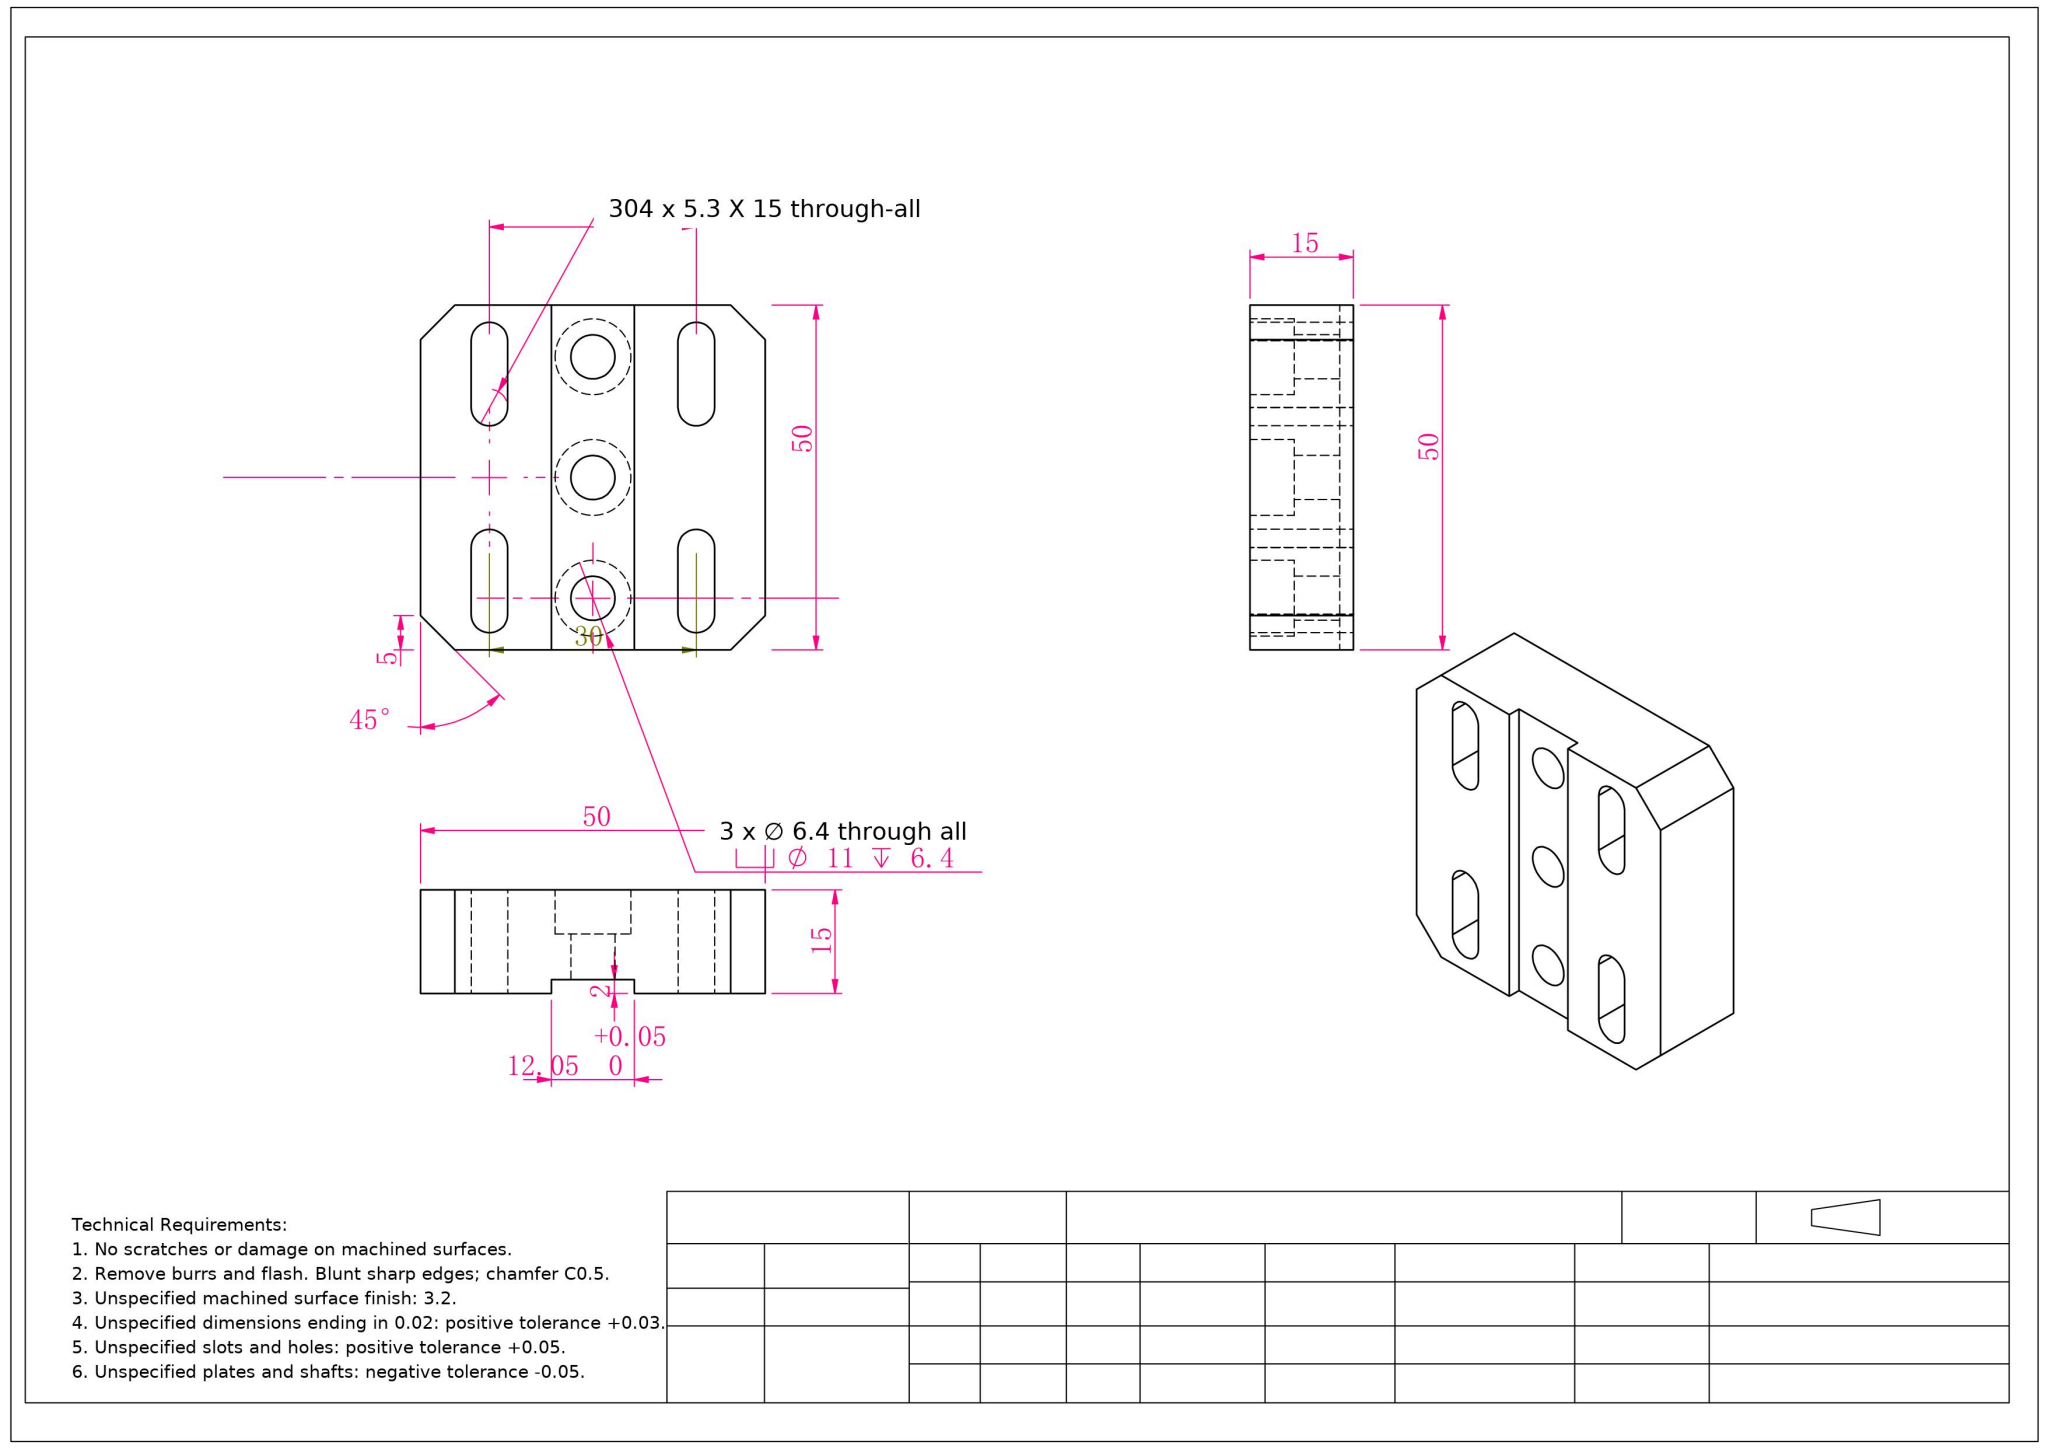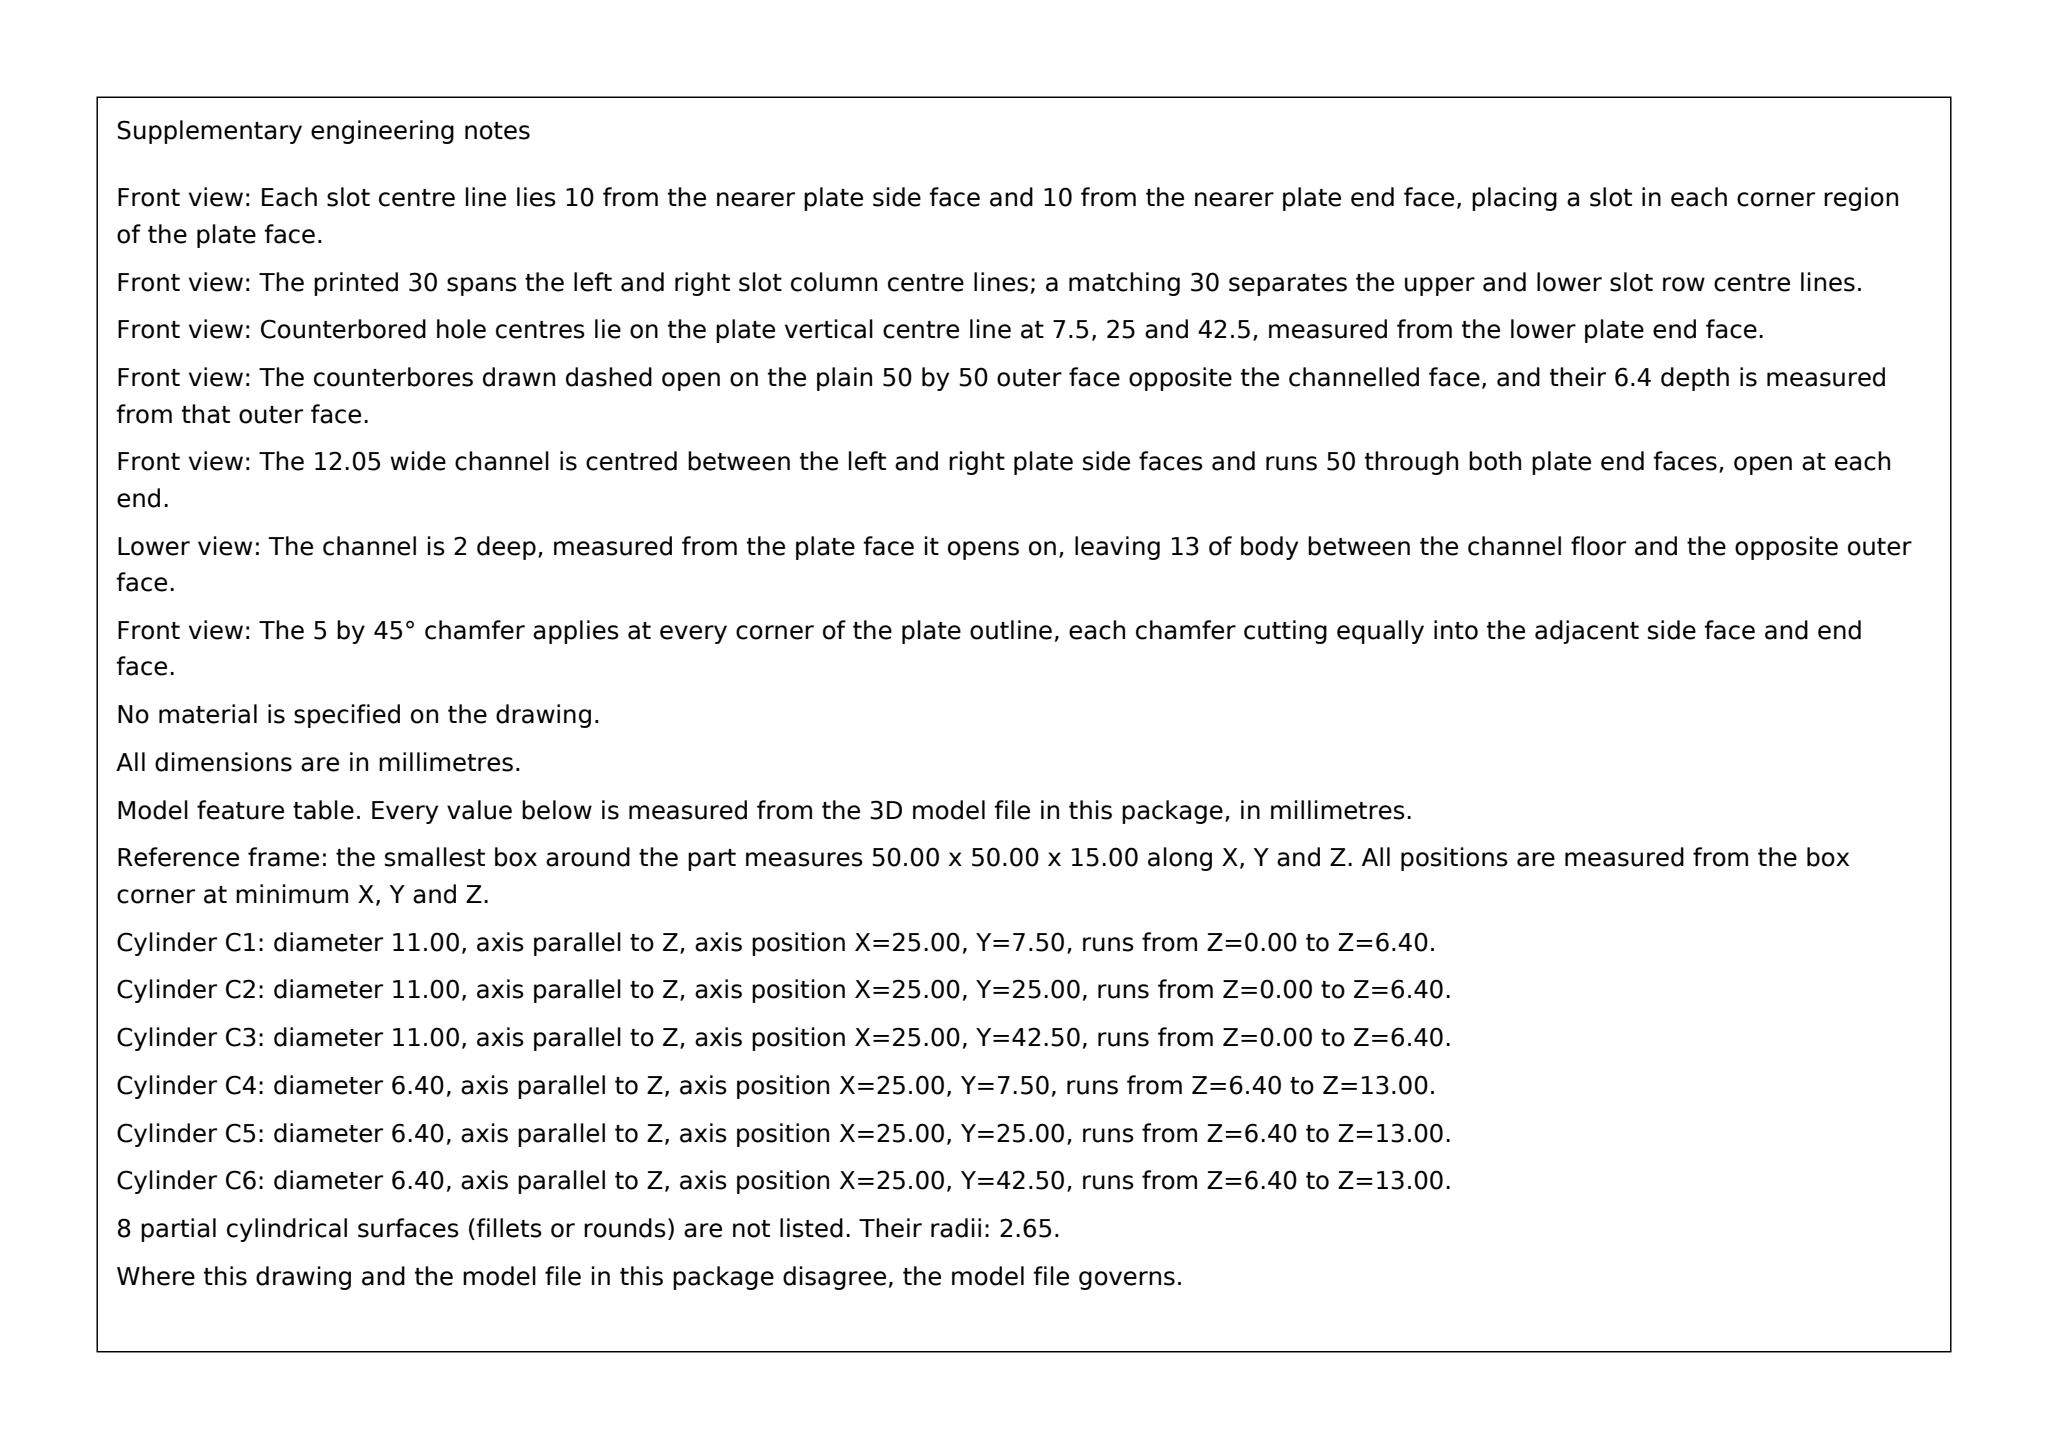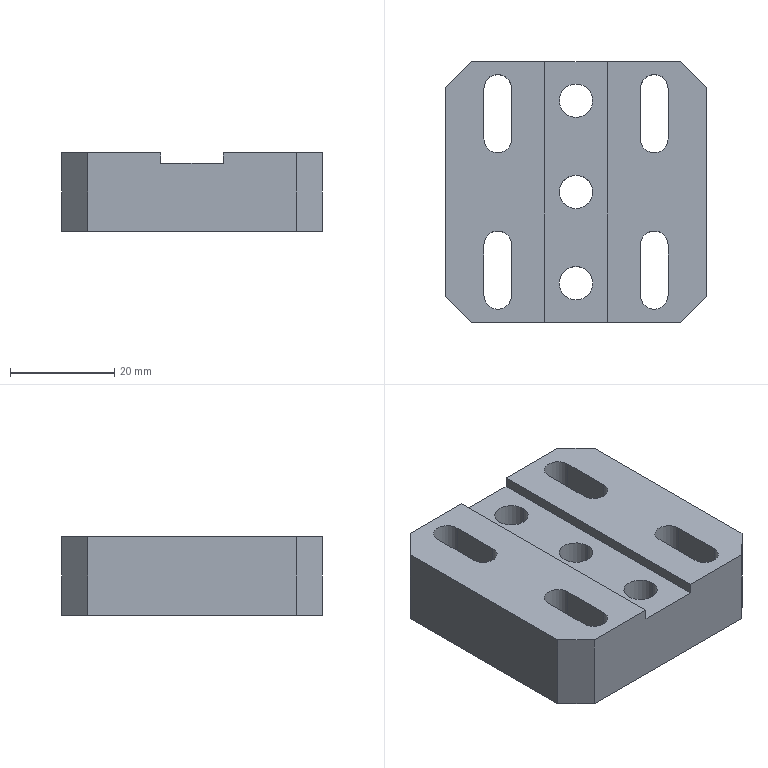Part | SolidWorks | mm | 1 solid | 45 faces | box 50 x 50 x 15 mm | volume 28675 mm3 | plane 25 | cylinder 20 | commonest cylinder face diameters 5.3 x8 11 x6 6.4 x6
Drawing notes:
4X SLOT 5.3 WIDE X 15 LG THRU ALL, SYM ABOUT BOTH CLS | from the solid: Ø5.3 z-cyls paired y=5.15/14.85 and 35.15/44.85 at x=10 & 40, len 15 thru plate
SLOT CLS 30 APART HORIZ AND 30 APART VERT | from the solid: slot centers x=10 & 40, y=10 & 40 in 50x50 bbox
3X Ø6.4 THRU ALL ON VERT CL (25 FROM EACH SIDE), 17.5 SPACING | from the solid: Ø6.4 z-cyls at x=25; y=7.5, 25.0, 42.5
END HOLES 7.5 FROM TOP/BOT EDGE, MID HOLE ON HORIZ CL | from the solid: hole y=7.5 and 42.5 in 50 height; y=25 on CL
3X CBORE Ø11 DP 6.4 FROM BACK FACE | from the solid: Ø11 len 6.4 + Ø6.4 len 6.6 = 13 of 15; z planes at 6.4 and 13
4X SLOT 5.3 WIDE X 15 LG THRU ALL; SLOT CLS AT X=10 AND X=40 FROM LEFT EDGE, SLOT END CENTRES AT Y=5.15/14.85 AND Y=35.15/44.85 FROM BOTTOM EDGE | from the solid: cylinders dia 5.3 axis z at (10,5.15),(10,14.85),(10,35.15),(10,44.85),(40,5.15),(40,14.85),(40,35.15),(40,44.85), length 15 = full thickness
FRONT FACE GROOVE 12.05 WIDE X 2 DEEP, FULL HEIGHT; GROOVE SIDES AT X=18.98 AND X=31.03 FROM LEFT EDGE (SYM ABOUT VERT CL) | from the solid: axis_planes x=18.98 and x=31.03 (width 12.05, centred on 25 of 50 bbox); z planes 13.0 and 15.0 (2 deep from front face)
3X Ø6.4 THRU ALL ON X=25 FROM LEFT EDGE, AT Y=7.5, 25.0, 42.5 FROM BOTTOM EDGE; CBORE Ø11 DP 6.4 FROM BACK FACE (Z=0) | from the solid: cylinders dia 6.4 at (25,7.5),(25,25),(25,42.5) len 6.6 and dia 11.0 same positions len 6.4; z plane 6.4
4X SLOT 5.3 WIDE X 15 LG, THRU ALL (15 THK); SLOT CLS AT 10 AND 40 FROM LEFT EDGE, 10 AND 40 FROM BOTTOM EDGE | from the solid: cylinders dia 5.3 axis z, length 15, at (10,5.15),(10,14.85),(10,35.15),(10,44.85),(40,5.15),(40,14.85),(40,35.15),(40,44.85)
FRONT-FACE GROOVE 12.05 WIDE X 2 DEEP, FULL HEIGHT; GROOVE FACES AT 18.98 AND 31.03 FROM LEFT EDGE (SYM ABOUT VERT CL) | from the solid: axis_planes x=18.98 and x=31.03 (12.05 apart, centred on 25 of 50 bbox); z=13.0 floor vs z=15.0 front face = 2 deep